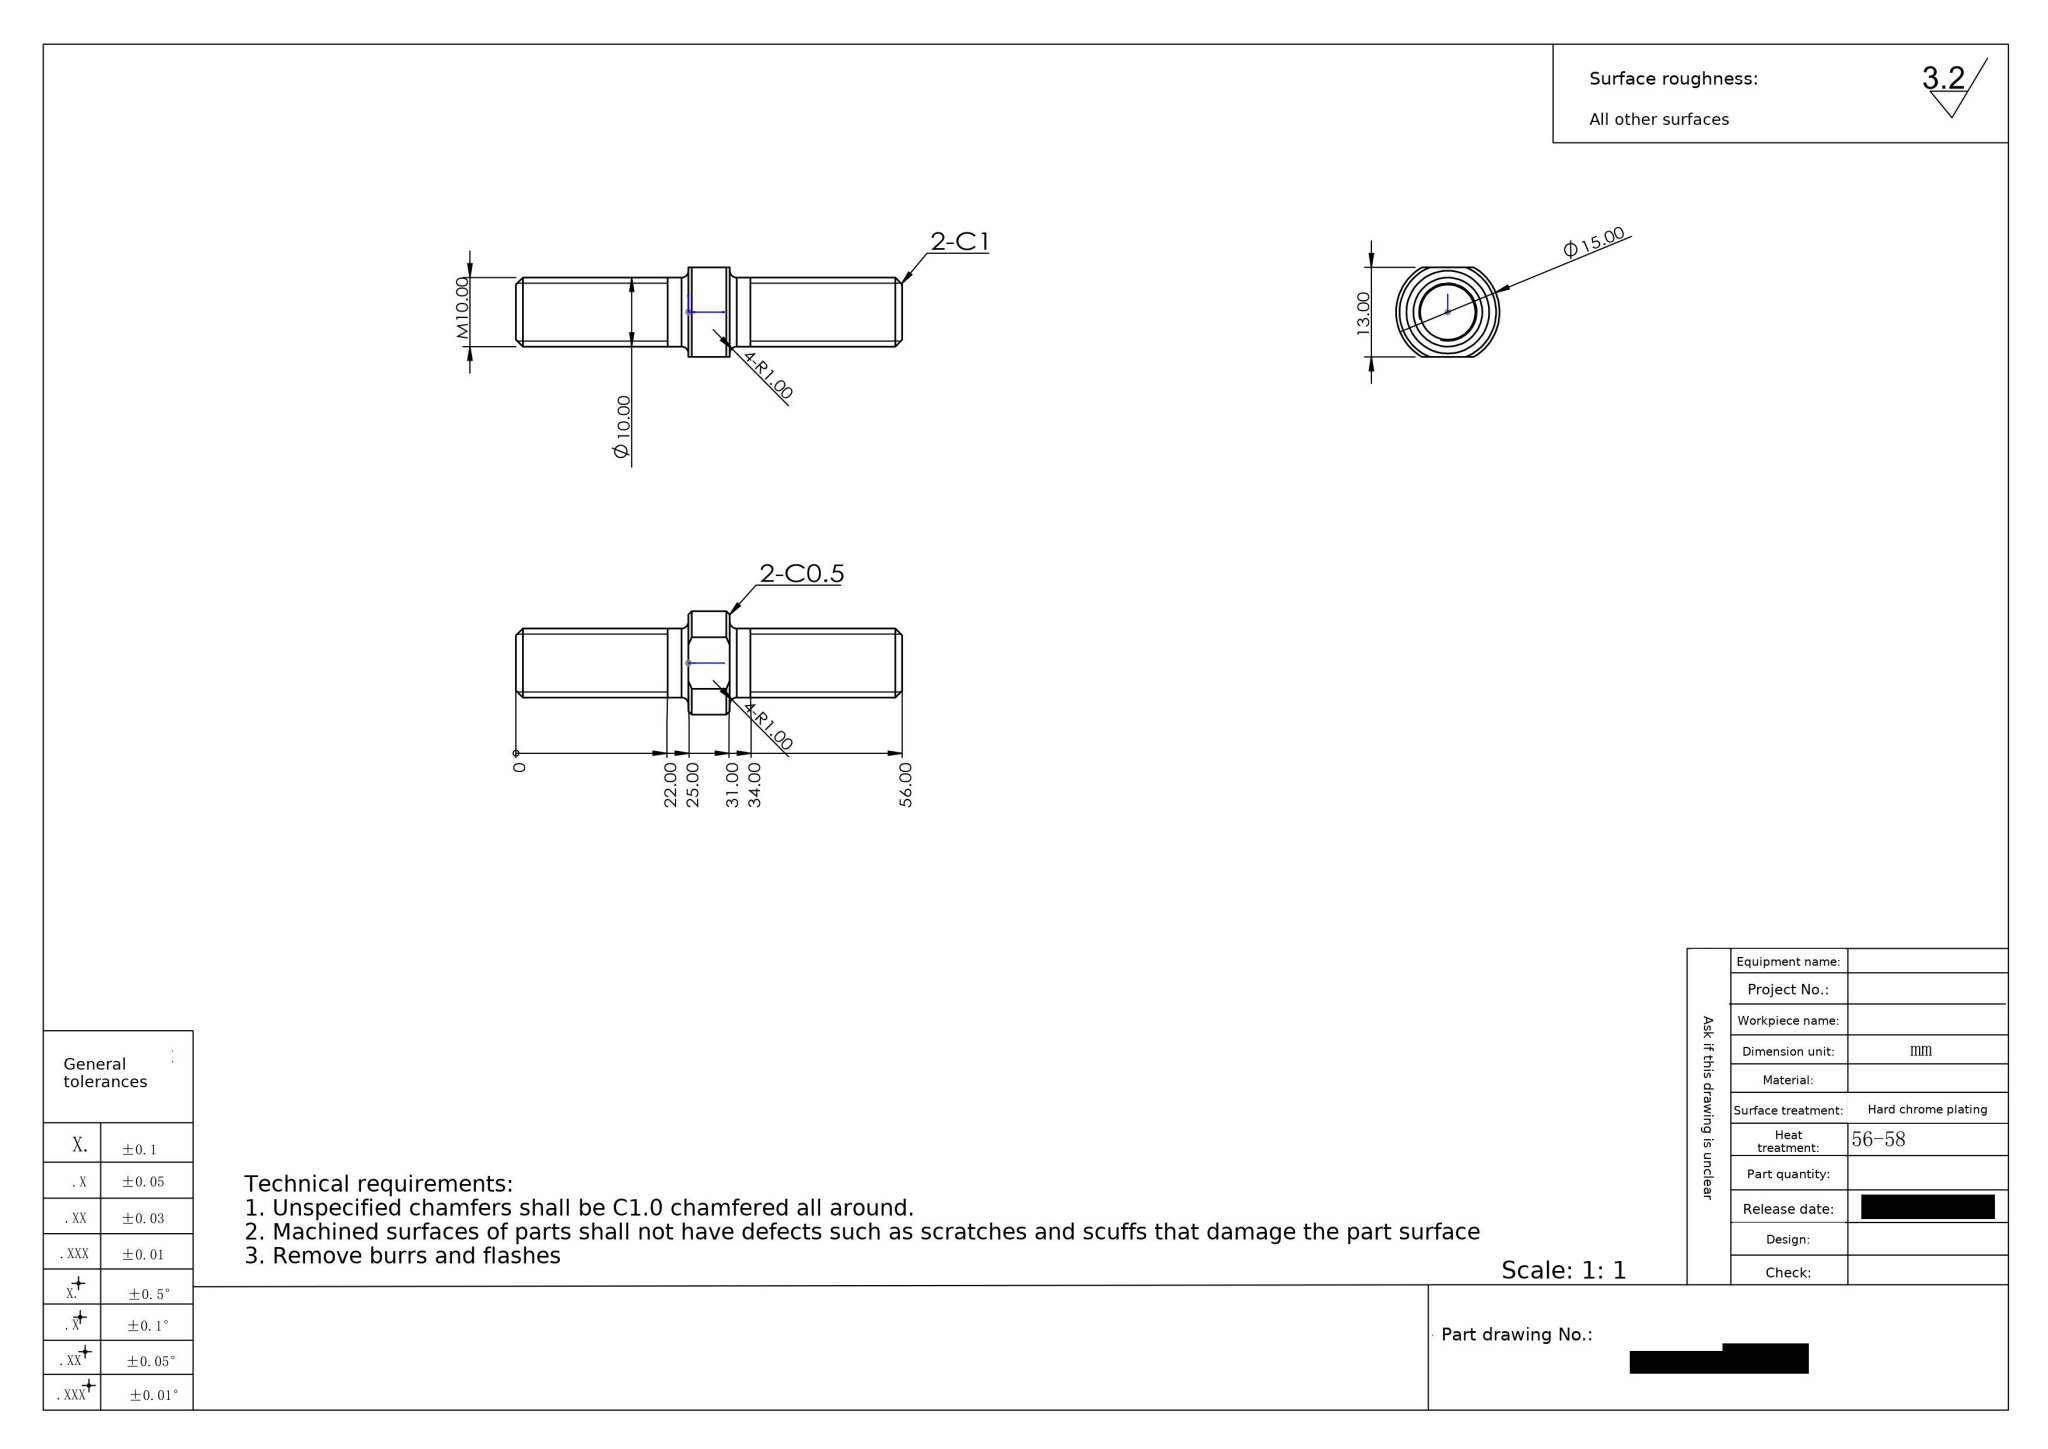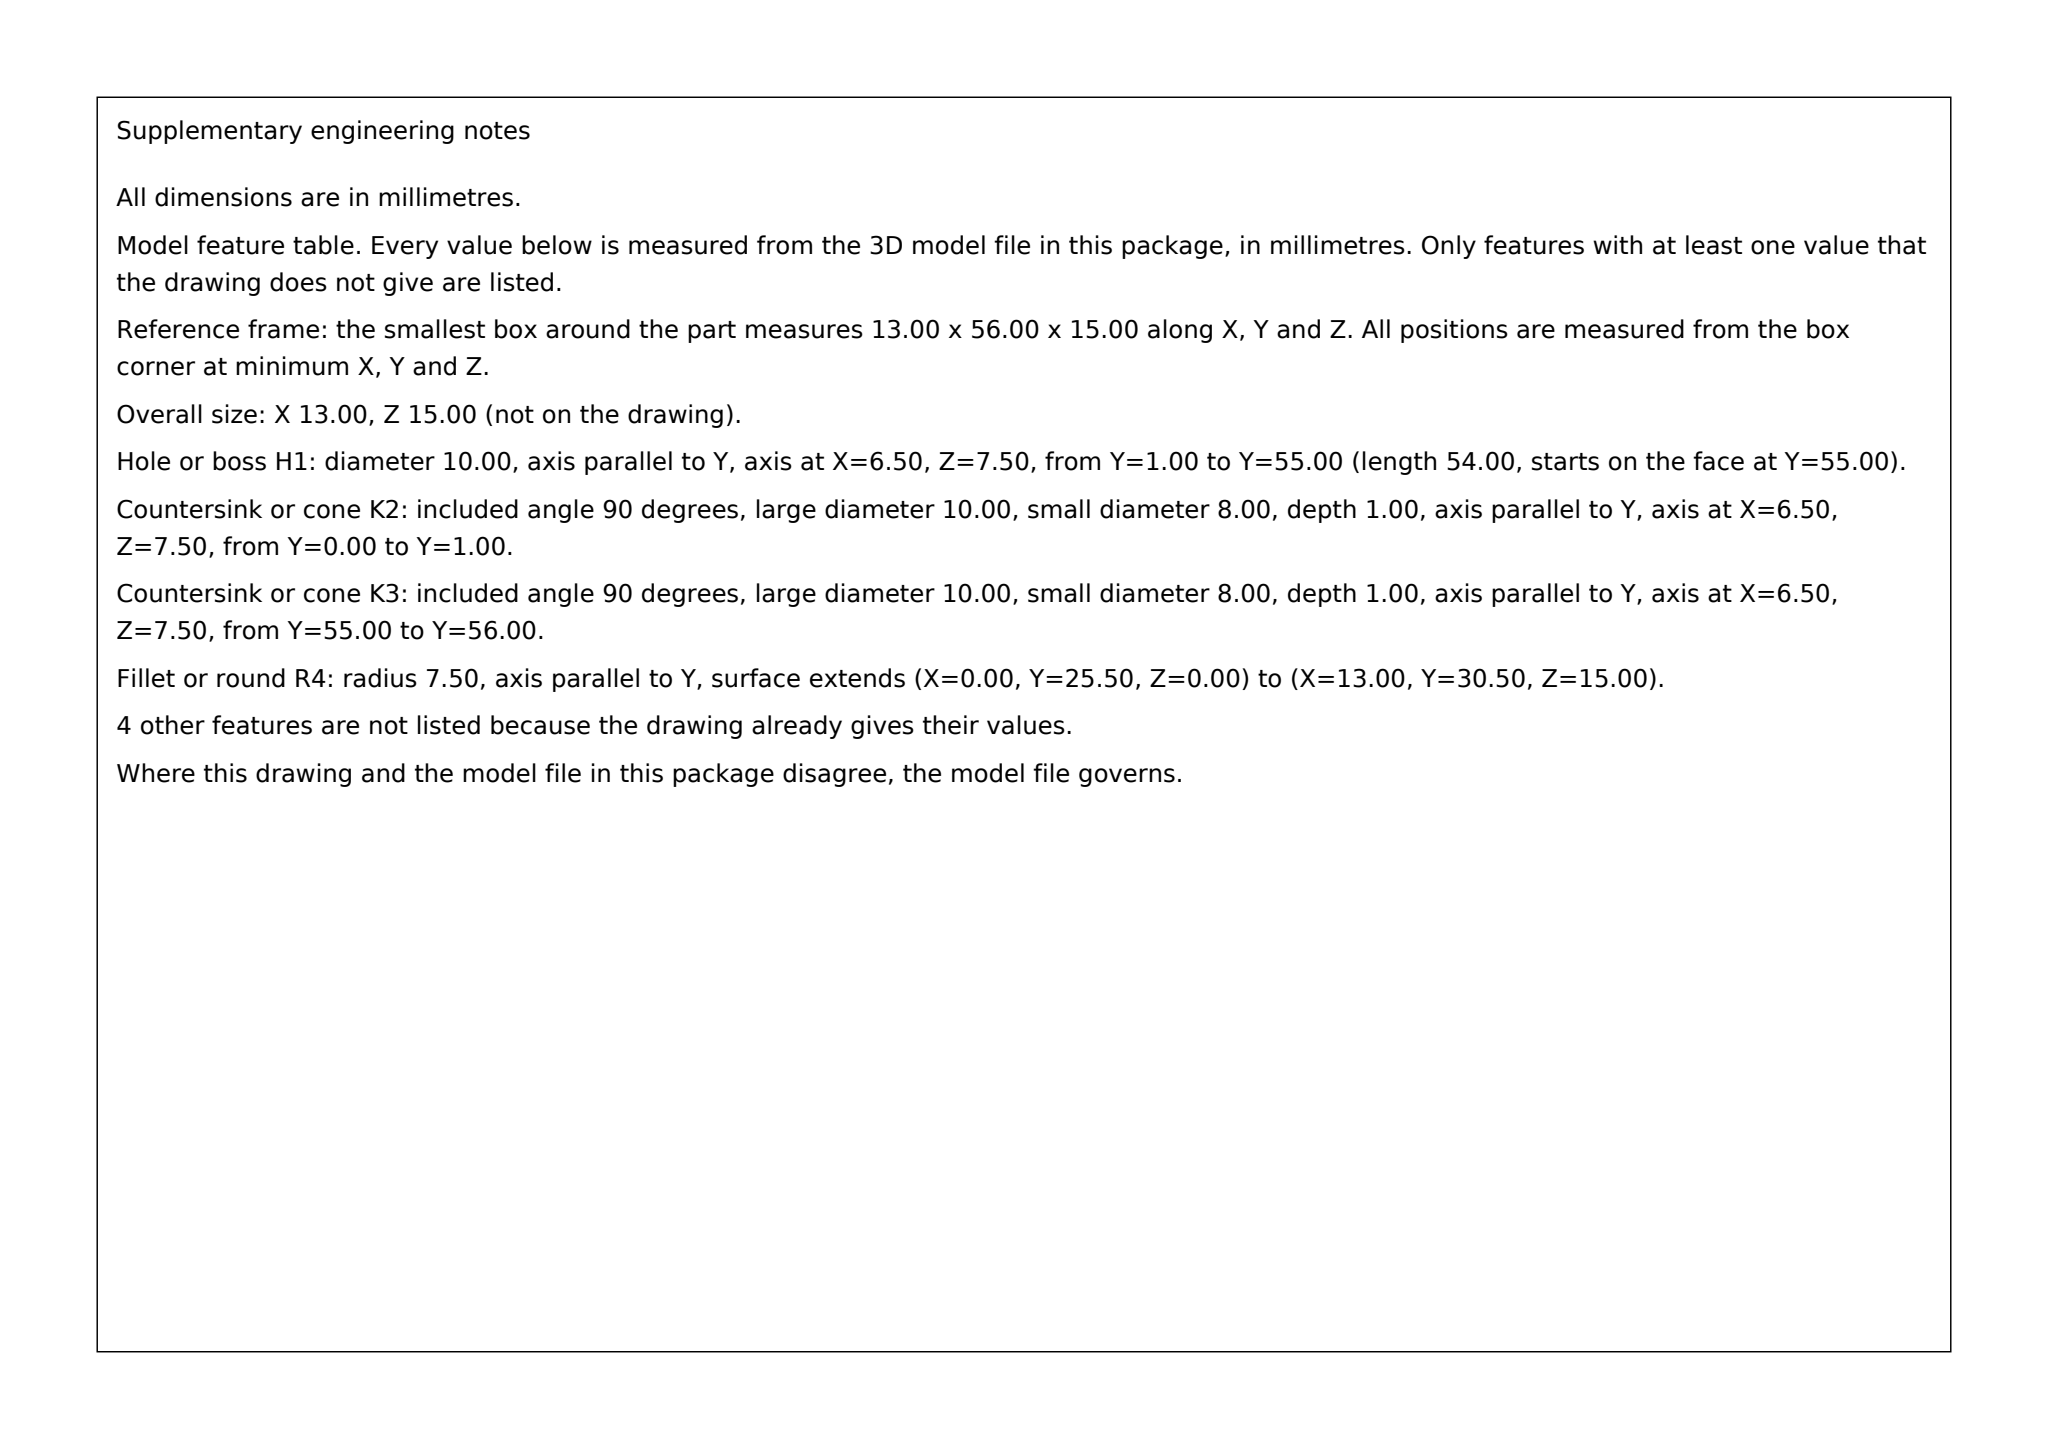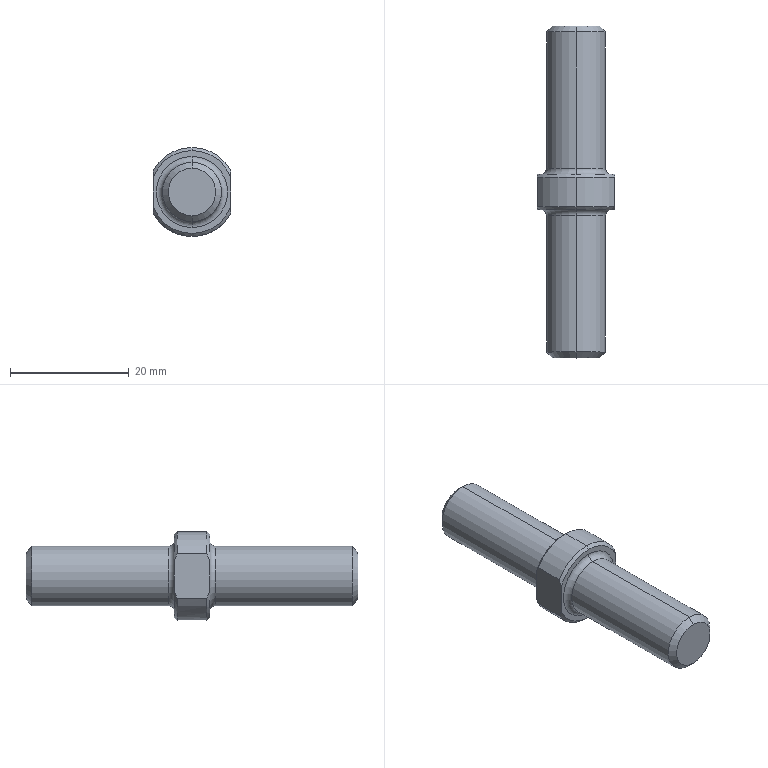Part | SolidWorks | mm | 1 solid | 27 faces | box 13 x 56 x 15 mm | volume 4903 mm3 | cone 10 | cylinder 7 | plane 6 | torus 4 | commonest cylinder face diameters 10 x4 15 x3
build123d program:
from build123d import *

# Parameters (mm, degrees)
CHAMFER1_SIZE      = 1
CUT_EXTRUDE1_DEPTH = 33.764
FILLET1_R          = 1
CHAMFER2_SIZE      = 0.5


with BuildPart() as part:
    # Sketch1 → Revolve1 (revolve)
    with BuildSketch(Plane.XY, mode=Mode.PRIVATE) as revolve1_sk:
        Polygon((0, -25), (5, -25), (5, 0), (7.5, 0), (7.5, 6), (5, 6), (5, 31), (0, 31), align=None)
    revolve(revolve1_sk.sketch.rotate(Axis((0, 36.907, 0), (0, -1, 0)), 90), axis=Axis((0, 36.907, 0), (0, -1, 0)))

    # Chamfer1
    chamfer1_edges = [part.edges().sort_by_distance(p)[0] for p in [
        (0, 31, -5),
        (0, -25, -5),
    ]]
    chamfer(chamfer1_edges, length=CHAMFER1_SIZE)

    # Sketch2 → Cut-Extrude1 (cut, through all)
    with BuildSketch(Plane(origin=(0, 6, 0), x_dir=(1, 0, 0), z_dir=(0, 1, 0))):
        with BuildLine():
            Line((-6.5, 3.742), (-6.5, -3.742))
            ThreePointArc((-6.5, -3.742), (-7.5, 0), (-6.5, 3.742))
        make_face()
        with BuildLine():
            Line((6.5, 3.742), (6.5, -3.742))
            ThreePointArc((6.5, -3.742), (7.5, 0), (6.5, 3.742))
        make_face()
    extrude(amount=-CUT_EXTRUDE1_DEPTH, mode=Mode.SUBTRACT)

    # Fillet1
    fillet1_edges = [part.edges().sort_by_distance(p)[0] for p in [
        (0, 6, -5),
        (0, 0, -5),
    ]]
    fillet(fillet1_edges, radius=FILLET1_R)

    # Chamfer2
    chamfer2_edges = [part.edges().sort_by_distance(p)[0] for p in [
        (0, 6, -7.5),
        (0, 0, -7.5),
        (0, 6, 7.5),
        (0, 0, 7.5),
    ]]
    chamfer(chamfer2_edges, length=CHAMFER2_SIZE)


solid = part.part
STEP:
#1=CARTESIAN_POINT('',(0.,0.,7.));
#2=VERTEX_POINT('',#1);
#3=CARTESIAN_POINT('',(-6.5,0.,2.598));
#4=VERTEX_POINT('',#3);
#5=CARTESIAN_POINT('',(0.,0.,0.));
#6=DIRECTION('',(0.,-1.,0.));
#7=DIRECTION('',(0.,0.,1.));
#8=AXIS2_PLACEMENT_3D('',#5,#6,#7);
#9=CIRCLE('',#8,7.);
#10=EDGE_CURVE('',#2,#4,#9,.T.);
#11=ORIENTED_EDGE('',*,*,#10,.F.);
#12=CARTESIAN_POINT('',(0.,0.5,7.5));
#13=VERTEX_POINT('',#12);
#14=CARTESIAN_POINT('',(0.,0.5,7.5));
#15=DIRECTION('',(0.,0.7071,0.7071));
#16=VECTOR('',#15,1000.);
#17=LINE('',#14,#16);
#18=EDGE_CURVE('',#2,#13,#17,.T.);
#19=ORIENTED_EDGE('',*,*,#18,.T.);
#20=CARTESIAN_POINT('',(-6.5,0.5,3.742));
#21=VERTEX_POINT('',#20);
#22=CARTESIAN_POINT('',(0.,0.5,0.));
#23=DIRECTION('',(0.,1.,0.));
#24=DIRECTION('',(0.,0.,1.));
#25=AXIS2_PLACEMENT_3D('',#22,#23,#24);
#26=CIRCLE('',#25,7.5);
#27=EDGE_CURVE('',#21,#13,#26,.T.);
#28=ORIENTED_EDGE('',*,*,#27,.F.);
#29=CARTESIAN_POINT('',(-6.5,0.,2.598));
#30=CARTESIAN_POINT('',(-6.5,0.145,2.989));
#31=CARTESIAN_POINT('',(-6.5,0.314,3.369));
#32=CARTESIAN_POINT('',(-6.5,0.5,3.742));
#33=B_SPLINE_CURVE_WITH_KNOTS('',3,(#29,#30,#31,#32),.UNSPECIFIED.,.F.,.F.,(4,4),(0.,0.001248),.UNSPECIFIED.);
#34=EDGE_CURVE('',#4,#21,#33,.T.);
#35=ORIENTED_EDGE('',*,*,#34,.F.);
#36=EDGE_LOOP('',(#11,#19,#28,#35));
#37=FACE_OUTER_BOUND('',#36,.T.);
#38=CARTESIAN_POINT('',(0.,0.5,0.));
#39=DIRECTION('',(0.,1.,0.));
#40=DIRECTION('',(0.,0.,1.));
#41=AXIS2_PLACEMENT_3D('',#38,#39,#40);
#42=CONICAL_SURFACE('',#41,7.5,0.7854);
#43=ADVANCED_FACE('',(#37),#42,.T.);
#44=CARTESIAN_POINT('',(0.,6.,-7.));
#45=VERTEX_POINT('',#44);
#46=CARTESIAN_POINT('',(-6.5,6.,-2.598));
#47=VERTEX_POINT('',#46);
#48=CARTESIAN_POINT('',(0.,6.,0.));
#49=DIRECTION('',(0.,1.,0.));
#50=DIRECTION('',(0.,0.,-1.));
#51=AXIS2_PLACEMENT_3D('',#48,#49,#50);
#52=CIRCLE('',#51,7.);
#53=EDGE_CURVE('',#45,#47,#52,.T.);
#54=ORIENTED_EDGE('',*,*,#53,.F.);
#55=CARTESIAN_POINT('',(0.,5.5,-7.5));
#56=VERTEX_POINT('',#55);
#57=CARTESIAN_POINT('',(0.,6.,-7.));
#58=DIRECTION('',(0.,-0.7071,-0.7071));
#59=VECTOR('',#58,1000.);
#60=LINE('',#57,#59);
#61=EDGE_CURVE('',#45,#56,#60,.T.);
#62=ORIENTED_EDGE('',*,*,#61,.T.);
#63=CARTESIAN_POINT('',(-6.5,5.5,-3.742));
#64=VERTEX_POINT('',#63);
#65=CARTESIAN_POINT('',(0.,5.5,0.));
#66=DIRECTION('',(0.,-1.,0.));
#67=DIRECTION('',(0.,0.,-1.));
#68=AXIS2_PLACEMENT_3D('',#65,#66,#67);
#69=CIRCLE('',#68,7.5);
#70=EDGE_CURVE('',#64,#56,#69,.T.);
#71=ORIENTED_EDGE('',*,*,#70,.F.);
#72=CARTESIAN_POINT('',(-6.5,6.,-2.598));
#73=CARTESIAN_POINT('',(-6.5,5.855,-2.989));
#74=CARTESIAN_POINT('',(-6.5,5.686,-3.369));
#75=CARTESIAN_POINT('',(-6.5,5.5,-3.742));
#76=B_SPLINE_CURVE_WITH_KNOTS('',3,(#72,#73,#74,#75),.UNSPECIFIED.,.F.,.F.,(4,4),(0.,0.001248),.UNSPECIFIED.);
#77=EDGE_CURVE('',#47,#64,#76,.T.);
#78=ORIENTED_EDGE('',*,*,#77,.F.);
#79=EDGE_LOOP('',(#54,#62,#71,#78));
#80=FACE_OUTER_BOUND('',#79,.T.);
#81=CARTESIAN_POINT('',(0.,6.,0.));
#82=DIRECTION('',(0.,-1.,0.));
#83=DIRECTION('',(0.,0.,-1.));
#84=AXIS2_PLACEMENT_3D('',#81,#82,#83);
#85=CONICAL_SURFACE('',#84,7.,0.7854);
#86=ADVANCED_FACE('',(#80),#85,.T.);
#87=CARTESIAN_POINT('',(0.,6.,6.));
#88=VERTEX_POINT('',#87);
#89=CARTESIAN_POINT('',(0.,6.,-6.));
#90=VERTEX_POINT('',#89);
#91=CARTESIAN_POINT('',(0.,6.,0.));
#92=DIRECTION('',(0.,-1.,0.));
#93=DIRECTION('',(0.,0.,-1.));
#94=AXIS2_PLACEMENT_3D('',#91,#92,#93);
#95=CIRCLE('',#94,6.);
#96=EDGE_CURVE('',#88,#90,#95,.T.);
#97=ORIENTED_EDGE('',*,*,#96,.F.);
#98=CARTESIAN_POINT('',(0.,7.,5.));
#99=VERTEX_POINT('',#98);
#100=CARTESIAN_POINT('',(0.,7.,6.));
#101=DIRECTION('',(1.,0.,-0.));
#102=DIRECTION('',(-0.,0.,-1.));
#103=AXIS2_PLACEMENT_3D('',#100,#101,#102);
#104=CIRCLE('',#103,1.);
#105=EDGE_CURVE('',#88,#99,#104,.T.);
#106=ORIENTED_EDGE('',*,*,#105,.T.);
#107=CARTESIAN_POINT('',(0.,7.,-5.));
#108=VERTEX_POINT('',#107);
#109=CARTESIAN_POINT('',(0.,7.,0.));
#110=DIRECTION('',(0.,1.,0.));
#111=DIRECTION('',(0.,0.,-1.));
#112=AXIS2_PLACEMENT_3D('',#109,#110,#111);
#113=CIRCLE('',#112,5.);
#114=EDGE_CURVE('',#108,#99,#113,.T.);
#115=ORIENTED_EDGE('',*,*,#114,.F.);
#116=CARTESIAN_POINT('',(0.,7.,-6.));
#117=DIRECTION('',(-1.,0.,0.));
#118=DIRECTION('',(0.,0.,1.));
#119=AXIS2_PLACEMENT_3D('',#116,#117,#118);
#120=CIRCLE('',#119,1.);
#121=EDGE_CURVE('',#90,#108,#120,.T.);
#122=ORIENTED_EDGE('',*,*,#121,.F.);
#123=EDGE_LOOP('',(#97,#106,#115,#122));
#124=FACE_OUTER_BOUND('',#123,.T.);
#125=CARTESIAN_POINT('',(0.,7.,0.));
#126=DIRECTION('',(0.,-1.,0.));
#127=DIRECTION('',(0.,0.,-1.));
#128=AXIS2_PLACEMENT_3D('',#125,#126,#127);
#129=TOROIDAL_SURFACE('',#128,6.,1.);
#130=ADVANCED_FACE('',(#124),#129,.F.);
#131=CARTESIAN_POINT('',(0.,-0.,-6.));
#132=VERTEX_POINT('',#131);
#133=CARTESIAN_POINT('',(0.,-0.,6.));
#134=VERTEX_POINT('',#133);
#135=CARTESIAN_POINT('',(0.,0.,0.));
#136=DIRECTION('',(0.,1.,0.));
#137=DIRECTION('',(0.,0.,1.));
#138=AXIS2_PLACEMENT_3D('',#135,#136,#137);
#139=CIRCLE('',#138,6.);
#140=EDGE_CURVE('',#132,#134,#139,.T.);
#141=ORIENTED_EDGE('',*,*,#140,.F.);
#142=CARTESIAN_POINT('',(0.,-1.,-5.));
#143=VERTEX_POINT('',#142);
#144=CARTESIAN_POINT('',(0.,-1.,-6.));
#145=DIRECTION('',(1.,0.,0.));
#146=DIRECTION('',(0.,0.,-1.));
#147=AXIS2_PLACEMENT_3D('',#144,#145,#146);
#148=CIRCLE('',#147,1.);
#149=EDGE_CURVE('',#132,#143,#148,.T.);
#150=ORIENTED_EDGE('',*,*,#149,.T.);
#151=CARTESIAN_POINT('',(0.,-1.,5.));
#152=VERTEX_POINT('',#151);
#153=CARTESIAN_POINT('',(0.,-1.,0.));
#154=DIRECTION('',(0.,-1.,0.));
#155=DIRECTION('',(0.,0.,1.));
#156=AXIS2_PLACEMENT_3D('',#153,#154,#155);
#157=CIRCLE('',#156,5.);
#158=EDGE_CURVE('',#152,#143,#157,.T.);
#159=ORIENTED_EDGE('',*,*,#158,.F.);
#160=CARTESIAN_POINT('',(0.,-1.,6.));
#161=DIRECTION('',(-1.,0.,0.));
#162=DIRECTION('',(0.,0.,1.));
#163=AXIS2_PLACEMENT_3D('',#160,#161,#162);
#164=CIRCLE('',#163,1.);
#165=EDGE_CURVE('',#134,#152,#164,.T.);
#166=ORIENTED_EDGE('',*,*,#165,.F.);
#167=EDGE_LOOP('',(#141,#150,#159,#166));
#168=FACE_OUTER_BOUND('',#167,.T.);
#169=CARTESIAN_POINT('',(0.,-1.,0.));
#170=DIRECTION('',(0.,1.,0.));
#171=DIRECTION('',(0.,0.,1.));
#172=AXIS2_PLACEMENT_3D('',#169,#170,#171);
#173=TOROIDAL_SURFACE('',#172,6.,1.);
#174=ADVANCED_FACE('',(#168),#173,.F.);
#175=CARTESIAN_POINT('',(0.,31.,4.));
#176=VERTEX_POINT('',#175);
#177=CARTESIAN_POINT('',(0.,31.,-4.));
#178=VERTEX_POINT('',#177);
#179=CARTESIAN_POINT('',(0.,31.,0.));
#180=DIRECTION('',(0.,1.,0.));
#181=DIRECTION('',(0.,0.,-1.));
#182=AXIS2_PLACEMENT_3D('',#179,#180,#181);
#183=CIRCLE('',#182,4.);
#184=EDGE_CURVE('',#176,#178,#183,.T.);
#185=ORIENTED_EDGE('',*,*,#184,.F.);
#186=CARTESIAN_POINT('',(0.,30.,5.));
#187=VERTEX_POINT('',#186);
#188=CARTESIAN_POINT('',(0.,31.,4.));
#189=DIRECTION('',(0.,-0.7071,0.7071));
#190=VECTOR('',#189,1000.);
#191=LINE('',#188,#190);
#192=EDGE_CURVE('',#176,#187,#191,.T.);
#193=ORIENTED_EDGE('',*,*,#192,.T.);
#194=CARTESIAN_POINT('',(0.,30.,-5.));
#195=VERTEX_POINT('',#194);
#196=CARTESIAN_POINT('',(0.,30.,0.));
#197=DIRECTION('',(0.,-1.,0.));
#198=DIRECTION('',(0.,0.,-1.));
#199=AXIS2_PLACEMENT_3D('',#196,#197,#198);
#200=CIRCLE('',#199,5.);
#201=EDGE_CURVE('',#195,#187,#200,.T.);
#202=ORIENTED_EDGE('',*,*,#201,.F.);
#203=CARTESIAN_POINT('',(0.,31.,-4.));
#204=DIRECTION('',(0.,-0.7071,-0.7071));
#205=VECTOR('',#204,1000.);
#206=LINE('',#203,#205);
#207=EDGE_CURVE('',#178,#195,#206,.T.);
#208=ORIENTED_EDGE('',*,*,#207,.F.);
#209=EDGE_LOOP('',(#185,#193,#202,#208));
#210=FACE_OUTER_BOUND('',#209,.T.);
#211=CARTESIAN_POINT('',(0.,31.,0.));
#212=DIRECTION('',(0.,-1.,0.));
#213=DIRECTION('',(0.,0.,-1.));
#214=AXIS2_PLACEMENT_3D('',#211,#212,#213);
#215=CONICAL_SURFACE('',#214,4.,0.7854);
#216=ADVANCED_FACE('',(#210),#215,.T.);
#217=CARTESIAN_POINT('',(0.,-25.,-4.));
#218=VERTEX_POINT('',#217);
#219=CARTESIAN_POINT('',(0.,-25.,4.));
#220=VERTEX_POINT('',#219);
#221=CARTESIAN_POINT('',(0.,-25.,0.));
#222=DIRECTION('',(0.,-1.,0.));
#223=DIRECTION('',(0.,0.,1.));
#224=AXIS2_PLACEMENT_3D('',#221,#222,#223);
#225=CIRCLE('',#224,4.);
#226=EDGE_CURVE('',#218,#220,#225,.T.);
#227=ORIENTED_EDGE('',*,*,#226,.F.);
#228=CARTESIAN_POINT('',(0.,-24.,-5.));
#229=VERTEX_POINT('',#228);
#230=CARTESIAN_POINT('',(0.,-24.,-5.));
#231=DIRECTION('',(0.,0.7071,-0.7071));
#232=VECTOR('',#231,1000.);
#233=LINE('',#230,#232);
#234=EDGE_CURVE('',#218,#229,#233,.T.);
#235=ORIENTED_EDGE('',*,*,#234,.T.);
#236=CARTESIAN_POINT('',(0.,-24.,5.));
#237=VERTEX_POINT('',#236);
#238=CARTESIAN_POINT('',(0.,-24.,0.));
#239=DIRECTION('',(0.,1.,0.));
#240=DIRECTION('',(0.,0.,1.));
#241=AXIS2_PLACEMENT_3D('',#238,#239,#240);
#242=CIRCLE('',#241,5.);
#243=EDGE_CURVE('',#237,#229,#242,.T.);
#244=ORIENTED_EDGE('',*,*,#243,.F.);
#245=CARTESIAN_POINT('',(0.,-24.,5.));
#246=DIRECTION('',(0.,0.7071,0.7071));
#247=VECTOR('',#246,1000.);
#248=LINE('',#245,#247);
#249=EDGE_CURVE('',#220,#237,#248,.T.);
#250=ORIENTED_EDGE('',*,*,#249,.F.);
#251=EDGE_LOOP('',(#227,#235,#244,#250));
#252=FACE_OUTER_BOUND('',#251,.T.);
#253=CARTESIAN_POINT('',(0.,-24.,0.));
#254=DIRECTION('',(0.,1.,0.));
#255=DIRECTION('',(0.,0.,1.));
#256=AXIS2_PLACEMENT_3D('',#253,#254,#255);
#257=CONICAL_SURFACE('',#256,5.,0.7854);
#258=ADVANCED_FACE('',(#252),#257,.T.);
#259=CARTESIAN_POINT('',(0.,7.,0.));
#260=DIRECTION('',(0.,1.,0.));
#261=DIRECTION('',(0.,0.,-1.));
#262=AXIS2_PLACEMENT_3D('',#259,#260,#261);
#263=CIRCLE('',#262,5.);
#264=EDGE_CURVE('',#99,#108,#263,.T.);
#265=ORIENTED_EDGE('',*,*,#264,.T.);
#266=CARTESIAN_POINT('',(0.,36.907,-5.));
#267=DIRECTION('',(0.,1.,0.));
#268=VECTOR('',#267,1000.);
#269=LINE('',#266,#268);
#270=EDGE_CURVE('',#108,#195,#269,.T.);
#271=ORIENTED_EDGE('',*,*,#270,.T.);
#272=ORIENTED_EDGE('',*,*,#201,.T.);
#273=CARTESIAN_POINT('',(0.,36.907,5.));
#274=DIRECTION('',(0.,1.,0.));
#275=VECTOR('',#274,1000.);
#276=LINE('',#273,#275);
#277=EDGE_CURVE('',#99,#187,#276,.T.);
#278=ORIENTED_EDGE('',*,*,#277,.F.);
#279=EDGE_LOOP('',(#265,#271,#272,#278));
#280=FACE_OUTER_BOUND('',#279,.T.);
#281=CARTESIAN_POINT('',(0.,36.907,0.));
#282=DIRECTION('',(0.,1.,0.));
#283=DIRECTION('',(0.,0.,1.));
#284=AXIS2_PLACEMENT_3D('',#281,#282,#283);
#285=CYLINDRICAL_SURFACE('',#284,5.);
#286=ADVANCED_FACE('',(#280),#285,.T.);
#287=ORIENTED_EDGE('',*,*,#27,.T.);
#288=CARTESIAN_POINT('',(0.,5.5,7.5));
#289=VERTEX_POINT('',#288);
#290=CARTESIAN_POINT('',(0.,36.907,7.5));
#291=DIRECTION('',(0.,1.,0.));
#292=VECTOR('',#291,1000.);
#293=LINE('',#290,#292);
#294=EDGE_CURVE('',#13,#289,#293,.T.);
#295=ORIENTED_EDGE('',*,*,#294,.T.);
#296=CARTESIAN_POINT('',(-6.5,5.5,3.742));
#297=VERTEX_POINT('',#296);
#298=CARTESIAN_POINT('',(0.,5.5,0.));
#299=DIRECTION('',(0.,-1.,0.));
#300=DIRECTION('',(0.,0.,-1.));
#301=AXIS2_PLACEMENT_3D('',#298,#299,#300);
#302=CIRCLE('',#301,7.5);
#303=EDGE_CURVE('',#289,#297,#302,.T.);
#304=ORIENTED_EDGE('',*,*,#303,.T.);
#305=CARTESIAN_POINT('',(-6.5,-25.,3.742));
#306=DIRECTION('',(0.,1.,0.));
#307=VECTOR('',#306,1000.);
#308=LINE('',#305,#307);
#309=EDGE_CURVE('',#21,#297,#308,.T.);
#310=ORIENTED_EDGE('',*,*,#309,.F.);
#311=EDGE_LOOP('',(#287,#295,#304,#310));
#312=FACE_OUTER_BOUND('',#311,.T.);
#313=CARTESIAN_POINT('',(0.,36.907,0.));
#314=DIRECTION('',(0.,1.,0.));
#315=DIRECTION('',(0.,0.,1.));
#316=AXIS2_PLACEMENT_3D('',#313,#314,#315);
#317=CYLINDRICAL_SURFACE('',#316,7.5);
#318=ADVANCED_FACE('',(#312),#317,.T.);
#319=ORIENTED_EDGE('',*,*,#243,.T.);
#320=CARTESIAN_POINT('',(0.,36.907,-5.));
#321=DIRECTION('',(0.,1.,0.));
#322=VECTOR('',#321,1000.);
#323=LINE('',#320,#322);
#324=EDGE_CURVE('',#229,#143,#323,.T.);
#325=ORIENTED_EDGE('',*,*,#324,.T.);
#326=CARTESIAN_POINT('',(0.,-1.,0.));
#327=DIRECTION('',(0.,-1.,0.));
#328=DIRECTION('',(0.,0.,1.));
#329=AXIS2_PLACEMENT_3D('',#326,#327,#328);
#330=CIRCLE('',#329,5.);
#331=EDGE_CURVE('',#143,#152,#330,.T.);
#332=ORIENTED_EDGE('',*,*,#331,.T.);
#333=CARTESIAN_POINT('',(0.,36.907,5.));
#334=DIRECTION('',(0.,1.,0.));
#335=VECTOR('',#334,1000.);
#336=LINE('',#333,#335);
#337=EDGE_CURVE('',#237,#152,#336,.T.);
#338=ORIENTED_EDGE('',*,*,#337,.F.);
#339=EDGE_LOOP('',(#319,#325,#332,#338));
#340=FACE_OUTER_BOUND('',#339,.T.);
#341=CARTESIAN_POINT('',(0.,36.907,0.));
#342=DIRECTION('',(0.,1.,0.));
#343=DIRECTION('',(0.,0.,1.));
#344=AXIS2_PLACEMENT_3D('',#341,#342,#343);
#345=CYLINDRICAL_SURFACE('',#344,5.);
#346=ADVANCED_FACE('',(#340),#345,.T.);
#347=CARTESIAN_POINT('',(6.5,0.5,-3.742));
#348=VERTEX_POINT('',#347);
#349=CARTESIAN_POINT('',(6.5,5.5,-3.742));
#350=VERTEX_POINT('',#349);
#351=CARTESIAN_POINT('',(6.5,-25.,-3.742));
#352=DIRECTION('',(0.,1.,0.));
#353=VECTOR('',#352,1000.);
#354=LINE('',#351,#353);
#355=EDGE_CURVE('',#348,#350,#354,.T.);
#356=ORIENTED_EDGE('',*,*,#355,.F.);
#357=CARTESIAN_POINT('',(-6.5,0.5,-3.742));
#358=VERTEX_POINT('',#357);
#359=CARTESIAN_POINT('',(0.,0.5,0.));
#360=DIRECTION('',(0.,1.,0.));
#361=DIRECTION('',(0.,0.,1.));
#362=AXIS2_PLACEMENT_3D('',#359,#360,#361);
#363=CIRCLE('',#362,7.5);
#364=EDGE_CURVE('',#348,#358,#363,.T.);
#365=ORIENTED_EDGE('',*,*,#364,.T.);
#366=CARTESIAN_POINT('',(-6.5,-25.,-3.742));
#367=DIRECTION('',(0.,1.,0.));
#368=VECTOR('',#367,1000.);
#369=LINE('',#366,#368);
#370=EDGE_CURVE('',#358,#64,#369,.T.);
#371=ORIENTED_EDGE('',*,*,#370,.T.);
#372=ORIENTED_EDGE('',*,*,#70,.T.);
#373=CARTESIAN_POINT('',(0.,5.5,0.));
#374=DIRECTION('',(0.,-1.,0.));
#375=DIRECTION('',(0.,0.,-1.));
#376=AXIS2_PLACEMENT_3D('',#373,#374,#375);
#377=CIRCLE('',#376,7.5);
#378=EDGE_CURVE('',#56,#350,#377,.T.);
#379=ORIENTED_EDGE('',*,*,#378,.T.);
#380=EDGE_LOOP('',(#356,#365,#371,#372,#379));
#381=FACE_OUTER_BOUND('',#380,.T.);
#382=CARTESIAN_POINT('',(0.,36.907,0.));
#383=DIRECTION('',(0.,1.,0.));
#384=DIRECTION('',(0.,0.,1.));
#385=AXIS2_PLACEMENT_3D('',#382,#383,#384);
#386=CYLINDRICAL_SURFACE('',#385,7.5);
#387=ADVANCED_FACE('',(#381),#386,.T.);
#388=CARTESIAN_POINT('',(0.,-25.,0.));
#389=DIRECTION('',(0.,-1.,0.));
#390=DIRECTION('',(0.,0.,1.));
#391=AXIS2_PLACEMENT_3D('',#388,#389,#390);
#392=CIRCLE('',#391,4.);
#393=EDGE_CURVE('',#220,#218,#392,.T.);
#394=ORIENTED_EDGE('',*,*,#393,.T.);
#395=ORIENTED_EDGE('',*,*,#226,.T.);
#396=EDGE_LOOP('',(#394,#395));
#397=FACE_OUTER_BOUND('',#396,.T.);
#398=CARTESIAN_POINT('',(0.,-25.,0.));
#399=DIRECTION('',(0.,1.,0.));
#400=DIRECTION('',(0.,0.,1.));
#401=AXIS2_PLACEMENT_3D('',#398,#399,#400);
#402=PLANE('',#401);
#403=ADVANCED_FACE('',(#397),#402,.F.);
#404=ORIENTED_EDGE('',*,*,#324,.F.);
#405=CARTESIAN_POINT('',(0.,-24.,0.));
#406=DIRECTION('',(0.,1.,0.));
#407=DIRECTION('',(0.,0.,1.));
#408=AXIS2_PLACEMENT_3D('',#405,#406,#407);
#409=CIRCLE('',#408,5.);
#410=EDGE_CURVE('',#229,#237,#409,.T.);
#411=ORIENTED_EDGE('',*,*,#410,.T.);
#412=ORIENTED_EDGE('',*,*,#337,.T.);
#413=ORIENTED_EDGE('',*,*,#158,.T.);
#414=EDGE_LOOP('',(#404,#411,#412,#413));
#415=FACE_OUTER_BOUND('',#414,.T.);
#416=CARTESIAN_POINT('',(0.,36.907,0.));
#417=DIRECTION('',(0.,1.,0.));
#418=DIRECTION('',(0.,0.,1.));
#419=AXIS2_PLACEMENT_3D('',#416,#417,#418);
#420=CYLINDRICAL_SURFACE('',#419,5.);
#421=ADVANCED_FACE('',(#415),#420,.T.);
#422=CARTESIAN_POINT('',(0.,0.,0.));
#423=DIRECTION('',(0.,1.,0.));
#424=DIRECTION('',(0.,0.,1.));
#425=AXIS2_PLACEMENT_3D('',#422,#423,#424);
#426=CIRCLE('',#425,6.);
#427=EDGE_CURVE('',#134,#132,#426,.T.);
#428=ORIENTED_EDGE('',*,*,#427,.T.);
#429=ORIENTED_EDGE('',*,*,#140,.T.);
#430=EDGE_LOOP('',(#428,#429));
#431=FACE_BOUND('',#430,.T.);
#432=CARTESIAN_POINT('',(-6.5,0.,-2.598));
#433=VERTEX_POINT('',#432);
#434=CARTESIAN_POINT('',(-6.5,0.,0.));
#435=DIRECTION('',(0.,0.,-1.));
#436=VECTOR('',#435,1000.);
#437=LINE('',#434,#436);
#438=EDGE_CURVE('',#4,#433,#437,.T.);
#439=ORIENTED_EDGE('',*,*,#438,.T.);
#440=CARTESIAN_POINT('',(6.5,0.,-2.598));
#441=VERTEX_POINT('',#440);
#442=CARTESIAN_POINT('',(0.,0.,0.));
#443=DIRECTION('',(0.,-1.,0.));
#444=DIRECTION('',(0.,0.,1.));
#445=AXIS2_PLACEMENT_3D('',#442,#443,#444);
#446=CIRCLE('',#445,7.);
#447=EDGE_CURVE('',#433,#441,#446,.T.);
#448=ORIENTED_EDGE('',*,*,#447,.T.);
#449=CARTESIAN_POINT('',(6.5,0.,2.598));
#450=VERTEX_POINT('',#449);
#451=CARTESIAN_POINT('',(6.5,0.,0.));
#452=DIRECTION('',(0.,0.,1.));
#453=VECTOR('',#452,1000.);
#454=LINE('',#451,#453);
#455=EDGE_CURVE('',#441,#450,#454,.T.);
#456=ORIENTED_EDGE('',*,*,#455,.T.);
#457=CARTESIAN_POINT('',(0.,0.,0.));
#458=DIRECTION('',(0.,-1.,0.));
#459=DIRECTION('',(-0.,0.,1.));
#460=AXIS2_PLACEMENT_3D('',#457,#458,#459);
#461=CIRCLE('',#460,7.);
#462=EDGE_CURVE('',#450,#2,#461,.T.);
#463=ORIENTED_EDGE('',*,*,#462,.T.);
#464=ORIENTED_EDGE('',*,*,#10,.T.);
#465=EDGE_LOOP('',(#439,#448,#456,#463,#464));
#466=FACE_OUTER_BOUND('',#465,.T.);
#467=CARTESIAN_POINT('',(5.,0.,0.));
#468=DIRECTION('',(0.,1.,0.));
#469=DIRECTION('',(0.,0.,1.));
#470=AXIS2_PLACEMENT_3D('',#467,#468,#469);
#471=PLANE('',#470);
#472=ADVANCED_FACE('',(#431,#466),#471,.F.);
#473=ORIENTED_EDGE('',*,*,#294,.F.);
#474=CARTESIAN_POINT('',(6.5,0.5,3.742));
#475=VERTEX_POINT('',#474);
#476=CARTESIAN_POINT('',(0.,0.5,0.));
#477=DIRECTION('',(0.,1.,0.));
#478=DIRECTION('',(0.,0.,1.));
#479=AXIS2_PLACEMENT_3D('',#476,#477,#478);
#480=CIRCLE('',#479,7.5);
#481=EDGE_CURVE('',#13,#475,#480,.T.);
#482=ORIENTED_EDGE('',*,*,#481,.T.);
#483=CARTESIAN_POINT('',(6.5,5.5,3.742));
#484=VERTEX_POINT('',#483);
#485=CARTESIAN_POINT('',(6.5,-25.,3.742));
#486=DIRECTION('',(0.,1.,0.));
#487=VECTOR('',#486,1000.);
#488=LINE('',#485,#487);
#489=EDGE_CURVE('',#475,#484,#488,.T.);
#490=ORIENTED_EDGE('',*,*,#489,.T.);
#491=CARTESIAN_POINT('',(0.,5.5,0.));
#492=DIRECTION('',(0.,-1.,0.));
#493=DIRECTION('',(0.,0.,-1.));
#494=AXIS2_PLACEMENT_3D('',#491,#492,#493);
#495=CIRCLE('',#494,7.5);
#496=EDGE_CURVE('',#484,#289,#495,.T.);
#497=ORIENTED_EDGE('',*,*,#496,.T.);
#498=EDGE_LOOP('',(#473,#482,#490,#497));
#499=FACE_OUTER_BOUND('',#498,.T.);
#500=CARTESIAN_POINT('',(0.,36.907,0.));
#501=DIRECTION('',(0.,1.,0.));
#502=DIRECTION('',(0.,0.,1.));
#503=AXIS2_PLACEMENT_3D('',#500,#501,#502);
#504=CYLINDRICAL_SURFACE('',#503,7.5);
#505=ADVANCED_FACE('',(#499),#504,.T.);
#506=CARTESIAN_POINT('',(0.,6.,0.));
#507=DIRECTION('',(0.,-1.,0.));
#508=DIRECTION('',(0.,0.,-1.));
#509=AXIS2_PLACEMENT_3D('',#506,#507,#508);
#510=CIRCLE('',#509,6.);
#511=EDGE_CURVE('',#90,#88,#510,.T.);
#512=ORIENTED_EDGE('',*,*,#511,.T.);
#513=ORIENTED_EDGE('',*,*,#96,.T.);
#514=EDGE_LOOP('',(#512,#513));
#515=FACE_BOUND('',#514,.T.);
#516=CARTESIAN_POINT('',(6.5,6.,-2.598));
#517=VERTEX_POINT('',#516);
#518=CARTESIAN_POINT('',(6.5,6.,2.598));
#519=VERTEX_POINT('',#518);
#520=CARTESIAN_POINT('',(6.5,6.,-3.742));
#521=DIRECTION('',(0.,0.,1.));
#522=VECTOR('',#521,1000.);
#523=LINE('',#520,#522);
#524=EDGE_CURVE('',#517,#519,#523,.T.);
#525=ORIENTED_EDGE('',*,*,#524,.F.);
#526=CARTESIAN_POINT('',(0.,6.,0.));
#527=DIRECTION('',(0.,1.,0.));
#528=DIRECTION('',(-0.,0.,-1.));
#529=AXIS2_PLACEMENT_3D('',#526,#527,#528);
#530=CIRCLE('',#529,7.);
#531=EDGE_CURVE('',#517,#45,#530,.T.);
#532=ORIENTED_EDGE('',*,*,#531,.T.);
#533=ORIENTED_EDGE('',*,*,#53,.T.);
#534=CARTESIAN_POINT('',(-6.5,6.,2.598));
#535=VERTEX_POINT('',#534);
#536=CARTESIAN_POINT('',(-6.5,6.,-3.742));
#537=DIRECTION('',(0.,0.,-1.));
#538=VECTOR('',#537,1000.);
#539=LINE('',#536,#538);
#540=EDGE_CURVE('',#535,#47,#539,.T.);
#541=ORIENTED_EDGE('',*,*,#540,.F.);
#542=CARTESIAN_POINT('',(0.,6.,0.));
#543=DIRECTION('',(0.,1.,0.));
#544=DIRECTION('',(0.,0.,-1.));
#545=AXIS2_PLACEMENT_3D('',#542,#543,#544);
#546=CIRCLE('',#545,7.);
#547=EDGE_CURVE('',#535,#519,#546,.T.);
#548=ORIENTED_EDGE('',*,*,#547,.T.);
#549=EDGE_LOOP('',(#525,#532,#533,#541,#548));
#550=FACE_OUTER_BOUND('',#549,.T.);
#551=CARTESIAN_POINT('',(7.5,6.,0.));
#552=DIRECTION('',(0.,-1.,0.));
#553=DIRECTION('',(0.,0.,-1.));
#554=AXIS2_PLACEMENT_3D('',#551,#552,#553);
#555=PLANE('',#554);
#556=ADVANCED_FACE('',(#515,#550),#555,.F.);
#557=ORIENTED_EDGE('',*,*,#270,.F.);
#558=ORIENTED_EDGE('',*,*,#114,.T.);
#559=ORIENTED_EDGE('',*,*,#277,.T.);
#560=CARTESIAN_POINT('',(0.,30.,0.));
#561=DIRECTION('',(0.,-1.,0.));
#562=DIRECTION('',(0.,0.,-1.));
#563=AXIS2_PLACEMENT_3D('',#560,#561,#562);
#564=CIRCLE('',#563,5.);
#565=EDGE_CURVE('',#187,#195,#564,.T.);
#566=ORIENTED_EDGE('',*,*,#565,.T.);
#567=EDGE_LOOP('',(#557,#558,#559,#566));
#568=FACE_OUTER_BOUND('',#567,.T.);
#569=CARTESIAN_POINT('',(0.,36.907,0.));
#570=DIRECTION('',(0.,1.,0.));
#571=DIRECTION('',(0.,0.,1.));
#572=AXIS2_PLACEMENT_3D('',#569,#570,#571);
#573=CYLINDRICAL_SURFACE('',#572,5.);
#574=ADVANCED_FACE('',(#568),#573,.T.);
#575=CARTESIAN_POINT('',(0.,31.,0.));
#576=DIRECTION('',(0.,1.,0.));
#577=DIRECTION('',(0.,0.,-1.));
#578=AXIS2_PLACEMENT_3D('',#575,#576,#577);
#579=CIRCLE('',#578,4.);
#580=EDGE_CURVE('',#178,#176,#579,.T.);
#581=ORIENTED_EDGE('',*,*,#580,.T.);
#582=ORIENTED_EDGE('',*,*,#184,.T.);
#583=EDGE_LOOP('',(#581,#582));
#584=FACE_OUTER_BOUND('',#583,.T.);
#585=CARTESIAN_POINT('',(5.,31.,0.));
#586=DIRECTION('',(0.,-1.,0.));
#587=DIRECTION('',(0.,0.,-1.));
#588=AXIS2_PLACEMENT_3D('',#585,#586,#587);
#589=PLANE('',#588);
#590=ADVANCED_FACE('',(#584),#589,.F.);
#591=ORIENTED_EDGE('',*,*,#234,.F.);
#592=ORIENTED_EDGE('',*,*,#393,.F.);
#593=ORIENTED_EDGE('',*,*,#249,.T.);
#594=ORIENTED_EDGE('',*,*,#410,.F.);
#595=EDGE_LOOP('',(#591,#592,#593,#594));
#596=FACE_OUTER_BOUND('',#595,.T.);
#597=CARTESIAN_POINT('',(0.,-24.,0.));
#598=DIRECTION('',(0.,1.,0.));
#599=DIRECTION('',(0.,0.,1.));
#600=AXIS2_PLACEMENT_3D('',#597,#598,#599);
#601=CONICAL_SURFACE('',#600,5.,0.7854);
#602=ADVANCED_FACE('',(#596),#601,.T.);
#603=ORIENTED_EDGE('',*,*,#192,.F.);
#604=ORIENTED_EDGE('',*,*,#580,.F.);
#605=ORIENTED_EDGE('',*,*,#207,.T.);
#606=ORIENTED_EDGE('',*,*,#565,.F.);
#607=EDGE_LOOP('',(#603,#604,#605,#606));
#608=FACE_OUTER_BOUND('',#607,.T.);
#609=CARTESIAN_POINT('',(0.,31.,0.));
#610=DIRECTION('',(0.,-1.,0.));
#611=DIRECTION('',(0.,0.,-1.));
#612=AXIS2_PLACEMENT_3D('',#609,#610,#611);
#613=CONICAL_SURFACE('',#612,4.,0.7854);
#614=ADVANCED_FACE('',(#608),#613,.T.);
#615=ORIENTED_EDGE('',*,*,#455,.F.);
#616=CARTESIAN_POINT('',(6.5,0.,-2.598));
#617=CARTESIAN_POINT('',(6.5,0.145,-2.989));
#618=CARTESIAN_POINT('',(6.5,0.314,-3.369));
#619=CARTESIAN_POINT('',(6.5,0.5,-3.742));
#620=B_SPLINE_CURVE_WITH_KNOTS('',3,(#616,#617,#618,#619),.UNSPECIFIED.,.F.,.F.,(4,4),(0.,0.001248),.UNSPECIFIED.);
#621=EDGE_CURVE('',#441,#348,#620,.T.);
#622=ORIENTED_EDGE('',*,*,#621,.T.);
#623=ORIENTED_EDGE('',*,*,#355,.T.);
#624=CARTESIAN_POINT('',(6.5,5.5,-3.742));
#625=CARTESIAN_POINT('',(6.5,5.686,-3.369));
#626=CARTESIAN_POINT('',(6.5,5.855,-2.989));
#627=CARTESIAN_POINT('',(6.5,6.,-2.598));
#628=B_SPLINE_CURVE_WITH_KNOTS('',3,(#624,#625,#626,#627),.UNSPECIFIED.,.F.,.F.,(4,4),(0.,0.001248),.UNSPECIFIED.);
#629=EDGE_CURVE('',#350,#517,#628,.T.);
#630=ORIENTED_EDGE('',*,*,#629,.T.);
#631=ORIENTED_EDGE('',*,*,#524,.T.);
#632=CARTESIAN_POINT('',(6.5,6.,2.598));
#633=CARTESIAN_POINT('',(6.5,5.855,2.989));
#634=CARTESIAN_POINT('',(6.5,5.686,3.369));
#635=CARTESIAN_POINT('',(6.5,5.5,3.742));
#636=B_SPLINE_CURVE_WITH_KNOTS('',3,(#632,#633,#634,#635),.UNSPECIFIED.,.F.,.F.,(4,4),(0.,0.001248),.UNSPECIFIED.);
#637=EDGE_CURVE('',#519,#484,#636,.T.);
#638=ORIENTED_EDGE('',*,*,#637,.T.);
#639=ORIENTED_EDGE('',*,*,#489,.F.);
#640=CARTESIAN_POINT('',(6.5,0.5,3.742));
#641=CARTESIAN_POINT('',(6.5,0.314,3.369));
#642=CARTESIAN_POINT('',(6.5,0.145,2.989));
#643=CARTESIAN_POINT('',(6.5,0.,2.598));
#644=B_SPLINE_CURVE_WITH_KNOTS('',3,(#640,#641,#642,#643),.UNSPECIFIED.,.F.,.F.,(4,4),(0.,0.001248),.UNSPECIFIED.);
#645=EDGE_CURVE('',#475,#450,#644,.T.);
#646=ORIENTED_EDGE('',*,*,#645,.T.);
#647=EDGE_LOOP('',(#615,#622,#623,#630,#631,#638,#639,#646));
#648=FACE_OUTER_BOUND('',#647,.T.);
#649=CARTESIAN_POINT('',(6.5,-25.,-3.742));
#650=DIRECTION('',(-1.,0.,0.));
#651=DIRECTION('',(0.,0.,1.));
#652=AXIS2_PLACEMENT_3D('',#649,#650,#651);
#653=PLANE('',#652);
#654=ADVANCED_FACE('',(#648),#653,.F.);
#655=ORIENTED_EDGE('',*,*,#370,.F.);
#656=CARTESIAN_POINT('',(-6.5,0.5,-3.742));
#657=CARTESIAN_POINT('',(-6.5,0.314,-3.369));
#658=CARTESIAN_POINT('',(-6.5,0.145,-2.989));
#659=CARTESIAN_POINT('',(-6.5,0.,-2.598));
#660=B_SPLINE_CURVE_WITH_KNOTS('',3,(#656,#657,#658,#659),.UNSPECIFIED.,.F.,.F.,(4,4),(0.,0.001248),.UNSPECIFIED.);
#661=EDGE_CURVE('',#358,#433,#660,.T.);
#662=ORIENTED_EDGE('',*,*,#661,.T.);
#663=ORIENTED_EDGE('',*,*,#438,.F.);
#664=ORIENTED_EDGE('',*,*,#34,.T.);
#665=ORIENTED_EDGE('',*,*,#309,.T.);
#666=CARTESIAN_POINT('',(-6.5,5.5,3.742));
#667=CARTESIAN_POINT('',(-6.5,5.686,3.369));
#668=CARTESIAN_POINT('',(-6.5,5.855,2.989));
#669=CARTESIAN_POINT('',(-6.5,6.,2.598));
#670=B_SPLINE_CURVE_WITH_KNOTS('',3,(#666,#667,#668,#669),.UNSPECIFIED.,.F.,.F.,(4,4),(0.,0.001248),.UNSPECIFIED.);
#671=EDGE_CURVE('',#297,#535,#670,.T.);
#672=ORIENTED_EDGE('',*,*,#671,.T.);
#673=ORIENTED_EDGE('',*,*,#540,.T.);
#674=ORIENTED_EDGE('',*,*,#77,.T.);
#675=EDGE_LOOP('',(#655,#662,#663,#664,#665,#672,#673,#674));
#676=FACE_OUTER_BOUND('',#675,.T.);
#677=CARTESIAN_POINT('',(-6.5,-25.,-3.742));
#678=DIRECTION('',(1.,0.,0.));
#679=DIRECTION('',(0.,0.,-1.));
#680=AXIS2_PLACEMENT_3D('',#677,#678,#679);
#681=PLANE('',#680);
#682=ADVANCED_FACE('',(#676),#681,.F.);
#683=ORIENTED_EDGE('',*,*,#149,.F.);
#684=ORIENTED_EDGE('',*,*,#427,.F.);
#685=ORIENTED_EDGE('',*,*,#165,.T.);
#686=ORIENTED_EDGE('',*,*,#331,.F.);
#687=EDGE_LOOP('',(#683,#684,#685,#686));
#688=FACE_OUTER_BOUND('',#687,.T.);
#689=CARTESIAN_POINT('',(0.,-1.,0.));
#690=DIRECTION('',(0.,1.,0.));
#691=DIRECTION('',(0.,0.,1.));
#692=AXIS2_PLACEMENT_3D('',#689,#690,#691);
#693=TOROIDAL_SURFACE('',#692,6.,1.);
#694=ADVANCED_FACE('',(#688),#693,.F.);
#695=ORIENTED_EDGE('',*,*,#105,.F.);
#696=ORIENTED_EDGE('',*,*,#511,.F.);
#697=ORIENTED_EDGE('',*,*,#121,.T.);
#698=ORIENTED_EDGE('',*,*,#264,.F.);
#699=EDGE_LOOP('',(#695,#696,#697,#698));
#700=FACE_OUTER_BOUND('',#699,.T.);
#701=CARTESIAN_POINT('',(0.,7.,0.));
#702=DIRECTION('',(0.,-1.,0.));
#703=DIRECTION('',(0.,0.,-1.));
#704=AXIS2_PLACEMENT_3D('',#701,#702,#703);
#705=TOROIDAL_SURFACE('',#704,6.,1.);
#706=ADVANCED_FACE('',(#700),#705,.F.);
#707=ORIENTED_EDGE('',*,*,#621,.F.);
#708=ORIENTED_EDGE('',*,*,#447,.F.);
#709=ORIENTED_EDGE('',*,*,#661,.F.);
#710=ORIENTED_EDGE('',*,*,#364,.F.);
#711=EDGE_LOOP('',(#707,#708,#709,#710));
#712=FACE_OUTER_BOUND('',#711,.T.);
#713=CARTESIAN_POINT('',(0.,0.5,0.));
#714=DIRECTION('',(0.,1.,0.));
#715=DIRECTION('',(0.,0.,1.));
#716=AXIS2_PLACEMENT_3D('',#713,#714,#715);
#717=CONICAL_SURFACE('',#716,7.5,0.7854);
#718=ADVANCED_FACE('',(#712),#717,.T.);
#719=ORIENTED_EDGE('',*,*,#61,.F.);
#720=ORIENTED_EDGE('',*,*,#531,.F.);
#721=ORIENTED_EDGE('',*,*,#629,.F.);
#722=ORIENTED_EDGE('',*,*,#378,.F.);
#723=EDGE_LOOP('',(#719,#720,#721,#722));
#724=FACE_OUTER_BOUND('',#723,.T.);
#725=CARTESIAN_POINT('',(0.,6.,0.));
#726=DIRECTION('',(0.,-1.,0.));
#727=DIRECTION('',(0.,0.,-1.));
#728=AXIS2_PLACEMENT_3D('',#725,#726,#727);
#729=CONICAL_SURFACE('',#728,7.,0.7854);
#730=ADVANCED_FACE('',(#724),#729,.T.);
#731=ORIENTED_EDGE('',*,*,#18,.F.);
#732=ORIENTED_EDGE('',*,*,#462,.F.);
#733=ORIENTED_EDGE('',*,*,#645,.F.);
#734=ORIENTED_EDGE('',*,*,#481,.F.);
#735=EDGE_LOOP('',(#731,#732,#733,#734));
#736=FACE_OUTER_BOUND('',#735,.T.);
#737=CARTESIAN_POINT('',(0.,0.5,0.));
#738=DIRECTION('',(0.,1.,0.));
#739=DIRECTION('',(0.,0.,1.));
#740=AXIS2_PLACEMENT_3D('',#737,#738,#739);
#741=CONICAL_SURFACE('',#740,7.5,0.7854);
#742=ADVANCED_FACE('',(#736),#741,.T.);
#743=ORIENTED_EDGE('',*,*,#671,.F.);
#744=ORIENTED_EDGE('',*,*,#303,.F.);
#745=ORIENTED_EDGE('',*,*,#496,.F.);
#746=ORIENTED_EDGE('',*,*,#637,.F.);
#747=ORIENTED_EDGE('',*,*,#547,.F.);
#748=EDGE_LOOP('',(#743,#744,#745,#746,#747));
#749=FACE_OUTER_BOUND('',#748,.T.);
#750=CARTESIAN_POINT('',(0.,6.,0.));
#751=DIRECTION('',(0.,-1.,0.));
#752=DIRECTION('',(0.,0.,-1.));
#753=AXIS2_PLACEMENT_3D('',#750,#751,#752);
#754=CONICAL_SURFACE('',#753,7.,0.7854);
#755=ADVANCED_FACE('',(#749),#754,.T.);
#756=CLOSED_SHELL('',(#43,#86,#130,#174,#216,#258,#286,#318,#346,#387,#403,#421,#472,#505,#556,#574,#590,#602,#614,#654,#682,#694,#706,#718,#730,#742,#755));
#757=MANIFOLD_SOLID_BREP('',#756);
#758=CARTESIAN_POINT('',(0.,0.,0.));
#759=DIRECTION('',(0.,0.,1.));
#760=DIRECTION('',(1.,0.,0.));
#761=AXIS2_PLACEMENT_3D('',#758,#759,#760);
#762=(LENGTH_UNIT()NAMED_UNIT(*)SI_UNIT(.MILLI.,.METRE.));
#763=UNCERTAINTY_MEASURE_WITH_UNIT(LENGTH_MEASURE(0.00001),#762,'','');
#764=(NAMED_UNIT(*)PLANE_ANGLE_UNIT()SI_UNIT($,.RADIAN.));
#765=(NAMED_UNIT(*)SI_UNIT($,.STERADIAN.)SOLID_ANGLE_UNIT());
#766=(GEOMETRIC_REPRESENTATION_CONTEXT(3)GLOBAL_UNCERTAINTY_ASSIGNED_CONTEXT((#763))GLOBAL_UNIT_ASSIGNED_CONTEXT((#762,#764,#765))REPRESENTATION_CONTEXT('',''));
#767=ADVANCED_BREP_SHAPE_REPRESENTATION('',(#757,#761),#766);